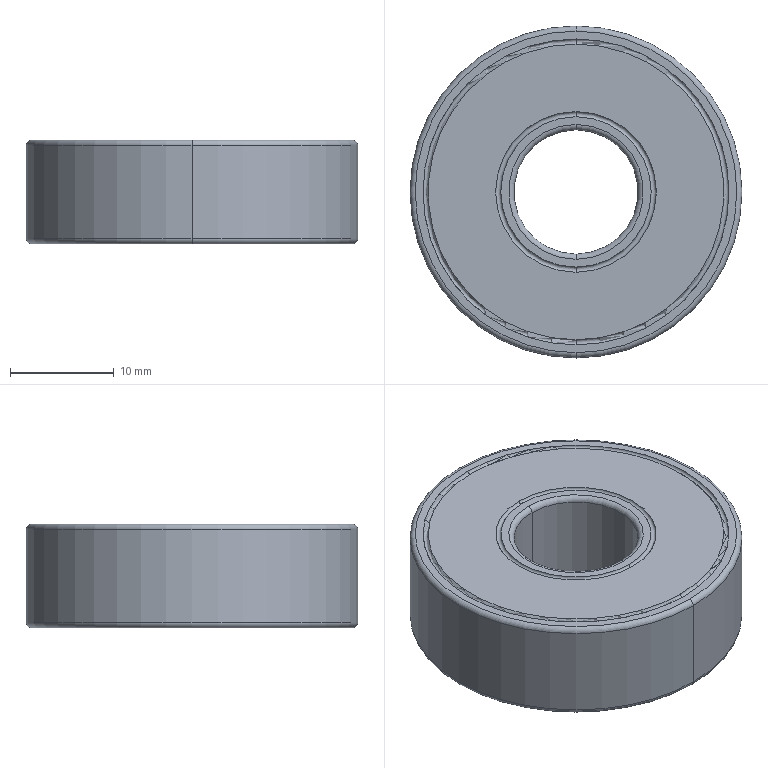Component | SolidWorks | --MA18S200416201Bearing-2 | 1 solid | 26 faces | box 32 x 32 x 10 mm | volume 6870 mm3 | torus 16 | plane 6 | cylinder 4 | commonest cylinder face diameters 12 x2 32 x2
build123d program:
from build123d import *

# Parameters (mm, degrees)
FILLET1_R = 0.5


with BuildPart() as part:
    # Sketch2 → Revolve1 (revolve)
    with BuildSketch(Plane.XY, mode=Mode.PRIVATE) as revolve1_sk:
        with BuildLine():
            Line((7.25, 10), (6, 10))
            Line((6, 10), (6, 0))
            Line((6, 0), (7.25, 0))
            ThreePointArc((7.25, 0), (7.5, 0.25), (7.75, 0))
            Line((7.75, 0), (14.25, 0))
            ThreePointArc((14.25, 0), (14.5, 0.25), (14.75, 0))
            Line((14.75, 0), (16, 0))
            Line((16, 0), (16, 10))
            Line((16, 10), (14.75, 10))
            ThreePointArc((14.75, 10), (14.5, 9.75), (14.25, 10))
            Line((14.25, 10), (7.75, 10))
            ThreePointArc((7.75, 10), (7.5, 9.75), (7.25, 10))
        make_face()
    revolve(revolve1_sk.sketch.rotate(Axis((0, 0, 0), (0, 1, 0)), 90), axis=Axis((0, 0, 0), (0, 1, 0)))

    # Fillet1
    fillet1_edges = [part.edges().sort_by_distance(p)[0] for p in [
        (0, 0, 6),
        (0, 10, 6),
        (0, 10, 16),
        (0, 0, 16),
    ]]
    fillet(fillet1_edges, radius=FILLET1_R)


solid = part.part

# Placed as in the assembly
solid = solid.moved(Location((72.885, -33.301, 50.5), (90, 0, 0)))
STEP:
#1=COLOUR_RGB('',0.7922,0.8196,0.9333);
#2=FILL_AREA_STYLE_COLOUR('',#1);
#3=FILL_AREA_STYLE('',(#2));
#4=SURFACE_STYLE_FILL_AREA(#3);
#5=SURFACE_SIDE_STYLE('',(#4));
#6=SURFACE_STYLE_USAGE(.BOTH.,#5);
#7=PRESENTATION_STYLE_ASSIGNMENT((#6));
#8=CARTESIAN_POINT('',(2.869,-1.941,2.008));
#9=VERTEX_POINT('',#8);
#10=CARTESIAN_POINT('',(2.869,-0.6811,2.008));
#11=VERTEX_POINT('',#10);
#12=CARTESIAN_POINT('',(2.869,-1.311,2.008));
#13=DIRECTION('',(0.,0.,1.));
#14=DIRECTION('',(0.,1.,0.));
#15=AXIS2_PLACEMENT_3D('',#12,#13,#14);
#16=CIRCLE('',#15,0.6299);
#17=EDGE_CURVE('',#9,#11,#16,.T.);
#18=ORIENTED_EDGE('',*,*,#17,.F.);
#19=CARTESIAN_POINT('',(2.869,-1.921,1.988));
#20=VERTEX_POINT('',#19);
#21=CARTESIAN_POINT('',(2.869,-1.921,2.008));
#22=DIRECTION('',(1.,0.,0.));
#23=DIRECTION('',(0.,1.,0.));
#24=AXIS2_PLACEMENT_3D('',#21,#22,#23);
#25=CIRCLE('',#24,0.01969);
#26=EDGE_CURVE('',#9,#20,#25,.T.);
#27=ORIENTED_EDGE('',*,*,#26,.T.);
#28=CARTESIAN_POINT('',(2.869,-0.7008,1.988));
#29=VERTEX_POINT('',#28);
#30=CARTESIAN_POINT('',(2.869,-1.311,1.988));
#31=DIRECTION('',(0.,0.,-1.));
#32=DIRECTION('',(0.,1.,0.));
#33=AXIS2_PLACEMENT_3D('',#30,#31,#32);
#34=CIRCLE('',#33,0.6102);
#35=EDGE_CURVE('',#29,#20,#34,.T.);
#36=ORIENTED_EDGE('',*,*,#35,.F.);
#37=CARTESIAN_POINT('',(2.869,-0.7008,2.008));
#38=DIRECTION('',(-1.,0.,0.));
#39=DIRECTION('',(0.,0.,1.));
#40=AXIS2_PLACEMENT_3D('',#37,#38,#39);
#41=CIRCLE('',#40,0.01969);
#42=EDGE_CURVE('',#11,#29,#41,.T.);
#43=ORIENTED_EDGE('',*,*,#42,.F.);
#44=EDGE_LOOP('',(#18,#27,#36,#43));
#45=FACE_OUTER_BOUND('',#44,.T.);
#46=CARTESIAN_POINT('',(2.869,-1.311,2.008));
#47=DIRECTION('',(0.,0.,-1.));
#48=DIRECTION('',(0.,1.,0.));
#49=AXIS2_PLACEMENT_3D('',#46,#47,#48);
#50=TOROIDAL_SURFACE('',#49,0.6102,0.01969);
#51=ADVANCED_FACE('',(#45),#50,.T.);
#52=CARTESIAN_POINT('',(2.869,-0.6811,2.362));
#53=VERTEX_POINT('',#52);
#54=CARTESIAN_POINT('',(2.869,-1.941,2.362));
#55=VERTEX_POINT('',#54);
#56=CARTESIAN_POINT('',(2.869,-1.311,2.362));
#57=DIRECTION('',(0.,0.,-1.));
#58=DIRECTION('',(0.,-1.,0.));
#59=AXIS2_PLACEMENT_3D('',#56,#57,#58);
#60=CIRCLE('',#59,0.6299);
#61=EDGE_CURVE('',#53,#55,#60,.T.);
#62=ORIENTED_EDGE('',*,*,#61,.F.);
#63=CARTESIAN_POINT('',(2.869,-0.7008,2.382));
#64=VERTEX_POINT('',#63);
#65=CARTESIAN_POINT('',(2.869,-0.7008,2.362));
#66=DIRECTION('',(1.,-0.,0.));
#67=DIRECTION('',(0.,1.,0.));
#68=AXIS2_PLACEMENT_3D('',#65,#66,#67);
#69=CIRCLE('',#68,0.01969);
#70=EDGE_CURVE('',#53,#64,#69,.T.);
#71=ORIENTED_EDGE('',*,*,#70,.T.);
#72=CARTESIAN_POINT('',(2.869,-1.921,2.382));
#73=VERTEX_POINT('',#72);
#74=CARTESIAN_POINT('',(2.869,-1.311,2.382));
#75=DIRECTION('',(0.,0.,1.));
#76=DIRECTION('',(0.,-1.,0.));
#77=AXIS2_PLACEMENT_3D('',#74,#75,#76);
#78=CIRCLE('',#77,0.6102);
#79=EDGE_CURVE('',#73,#64,#78,.T.);
#80=ORIENTED_EDGE('',*,*,#79,.F.);
#81=CARTESIAN_POINT('',(2.869,-1.921,2.362));
#82=DIRECTION('',(-1.,0.,0.));
#83=DIRECTION('',(0.,0.,1.));
#84=AXIS2_PLACEMENT_3D('',#81,#82,#83);
#85=CIRCLE('',#84,0.01969);
#86=EDGE_CURVE('',#55,#73,#85,.T.);
#87=ORIENTED_EDGE('',*,*,#86,.F.);
#88=EDGE_LOOP('',(#62,#71,#80,#87));
#89=FACE_OUTER_BOUND('',#88,.T.);
#90=CARTESIAN_POINT('',(2.869,-1.311,2.362));
#91=DIRECTION('',(0.,0.,1.));
#92=DIRECTION('',(0.,-1.,0.));
#93=AXIS2_PLACEMENT_3D('',#90,#91,#92);
#94=TOROIDAL_SURFACE('',#93,0.6102,0.01969);
#95=ADVANCED_FACE('',(#89),#94,.T.);
#96=CARTESIAN_POINT('',(2.869,-1.567,1.988));
#97=VERTEX_POINT('',#96);
#98=CARTESIAN_POINT('',(2.869,-1.055,1.988));
#99=VERTEX_POINT('',#98);
#100=CARTESIAN_POINT('',(2.869,-1.311,1.988));
#101=DIRECTION('',(0.,0.,1.));
#102=DIRECTION('',(0.,1.,0.));
#103=AXIS2_PLACEMENT_3D('',#100,#101,#102);
#104=CIRCLE('',#103,0.2559);
#105=EDGE_CURVE('',#97,#99,#104,.T.);
#106=ORIENTED_EDGE('',*,*,#105,.F.);
#107=CARTESIAN_POINT('',(2.869,-1.547,2.008));
#108=VERTEX_POINT('',#107);
#109=CARTESIAN_POINT('',(2.869,-1.567,2.008));
#110=DIRECTION('',(1.,0.,0.));
#111=DIRECTION('',(0.,1.,0.));
#112=AXIS2_PLACEMENT_3D('',#109,#110,#111);
#113=CIRCLE('',#112,0.01969);
#114=EDGE_CURVE('',#97,#108,#113,.T.);
#115=ORIENTED_EDGE('',*,*,#114,.T.);
#116=CARTESIAN_POINT('',(2.869,-1.075,2.008));
#117=VERTEX_POINT('',#116);
#118=CARTESIAN_POINT('',(2.869,-1.311,2.008));
#119=DIRECTION('',(0.,0.,-1.));
#120=DIRECTION('',(0.,1.,0.));
#121=AXIS2_PLACEMENT_3D('',#118,#119,#120);
#122=CIRCLE('',#121,0.2362);
#123=EDGE_CURVE('',#117,#108,#122,.T.);
#124=ORIENTED_EDGE('',*,*,#123,.F.);
#125=CARTESIAN_POINT('',(2.869,-1.055,2.008));
#126=DIRECTION('',(-1.,0.,0.));
#127=DIRECTION('',(0.,0.,1.));
#128=AXIS2_PLACEMENT_3D('',#125,#126,#127);
#129=CIRCLE('',#128,0.01969);
#130=EDGE_CURVE('',#99,#117,#129,.T.);
#131=ORIENTED_EDGE('',*,*,#130,.F.);
#132=EDGE_LOOP('',(#106,#115,#124,#131));
#133=FACE_OUTER_BOUND('',#132,.T.);
#134=CARTESIAN_POINT('',(2.869,-1.311,2.008));
#135=DIRECTION('',(0.,0.,-1.));
#136=DIRECTION('',(0.,1.,0.));
#137=AXIS2_PLACEMENT_3D('',#134,#135,#136);
#138=TOROIDAL_SURFACE('',#137,0.2559,0.01969);
#139=ADVANCED_FACE('',(#133),#138,.T.);
#140=CARTESIAN_POINT('',(2.869,-1.055,2.382));
#141=VERTEX_POINT('',#140);
#142=CARTESIAN_POINT('',(2.869,-1.567,2.382));
#143=VERTEX_POINT('',#142);
#144=CARTESIAN_POINT('',(2.869,-1.311,2.382));
#145=DIRECTION('',(0.,0.,-1.));
#146=DIRECTION('',(0.,-1.,0.));
#147=AXIS2_PLACEMENT_3D('',#144,#145,#146);
#148=CIRCLE('',#147,0.2559);
#149=EDGE_CURVE('',#141,#143,#148,.T.);
#150=ORIENTED_EDGE('',*,*,#149,.F.);
#151=CARTESIAN_POINT('',(2.869,-1.075,2.362));
#152=VERTEX_POINT('',#151);
#153=CARTESIAN_POINT('',(2.869,-1.055,2.362));
#154=DIRECTION('',(1.,-0.,0.));
#155=DIRECTION('',(0.,1.,0.));
#156=AXIS2_PLACEMENT_3D('',#153,#154,#155);
#157=CIRCLE('',#156,0.01969);
#158=EDGE_CURVE('',#141,#152,#157,.T.);
#159=ORIENTED_EDGE('',*,*,#158,.T.);
#160=CARTESIAN_POINT('',(2.869,-1.547,2.362));
#161=VERTEX_POINT('',#160);
#162=CARTESIAN_POINT('',(2.869,-1.311,2.362));
#163=DIRECTION('',(0.,0.,1.));
#164=DIRECTION('',(0.,-1.,0.));
#165=AXIS2_PLACEMENT_3D('',#162,#163,#164);
#166=CIRCLE('',#165,0.2362);
#167=EDGE_CURVE('',#161,#152,#166,.T.);
#168=ORIENTED_EDGE('',*,*,#167,.F.);
#169=CARTESIAN_POINT('',(2.869,-1.567,2.362));
#170=DIRECTION('',(-1.,0.,0.));
#171=DIRECTION('',(0.,0.,1.));
#172=AXIS2_PLACEMENT_3D('',#169,#170,#171);
#173=CIRCLE('',#172,0.01969);
#174=EDGE_CURVE('',#143,#161,#173,.T.);
#175=ORIENTED_EDGE('',*,*,#174,.F.);
#176=EDGE_LOOP('',(#150,#159,#168,#175));
#177=FACE_OUTER_BOUND('',#176,.T.);
#178=CARTESIAN_POINT('',(2.869,-1.311,2.362));
#179=DIRECTION('',(0.,0.,1.));
#180=DIRECTION('',(0.,-1.,0.));
#181=AXIS2_PLACEMENT_3D('',#178,#179,#180);
#182=TOROIDAL_SURFACE('',#181,0.2559,0.01969);
#183=ADVANCED_FACE('',(#177),#182,.T.);
#184=CARTESIAN_POINT('',(2.869,-0.75,2.382));
#185=VERTEX_POINT('',#184);
#186=CARTESIAN_POINT('',(2.869,-1.872,2.382));
#187=VERTEX_POINT('',#186);
#188=CARTESIAN_POINT('',(2.869,-1.311,2.382));
#189=DIRECTION('',(0.,0.,1.));
#190=DIRECTION('',(0.,-1.,0.));
#191=AXIS2_PLACEMENT_3D('',#188,#189,#190);
#192=CIRCLE('',#191,0.561);
#193=EDGE_CURVE('',#185,#187,#192,.T.);
#194=ORIENTED_EDGE('',*,*,#193,.F.);
#195=CARTESIAN_POINT('',(2.869,-0.7304,2.382));
#196=VERTEX_POINT('',#195);
#197=CARTESIAN_POINT('',(2.869,-0.7402,2.382));
#198=DIRECTION('',(1.,-0.,0.));
#199=DIRECTION('',(0.,1.,0.));
#200=AXIS2_PLACEMENT_3D('',#197,#198,#199);
#201=CIRCLE('',#200,0.009843);
#202=EDGE_CURVE('',#185,#196,#201,.T.);
#203=ORIENTED_EDGE('',*,*,#202,.T.);
#204=CARTESIAN_POINT('',(2.869,-1.892,2.382));
#205=VERTEX_POINT('',#204);
#206=CARTESIAN_POINT('',(2.869,-1.311,2.382));
#207=DIRECTION('',(0.,0.,1.));
#208=DIRECTION('',(0.,-1.,0.));
#209=AXIS2_PLACEMENT_3D('',#206,#207,#208);
#210=CIRCLE('',#209,0.5807);
#211=EDGE_CURVE('',#196,#205,#210,.T.);
#212=ORIENTED_EDGE('',*,*,#211,.T.);
#213=CARTESIAN_POINT('',(2.869,-1.882,2.382));
#214=DIRECTION('',(-1.,0.,0.));
#215=DIRECTION('',(0.,0.,1.));
#216=AXIS2_PLACEMENT_3D('',#213,#214,#215);
#217=CIRCLE('',#216,0.009843);
#218=EDGE_CURVE('',#187,#205,#217,.T.);
#219=ORIENTED_EDGE('',*,*,#218,.F.);
#220=EDGE_LOOP('',(#194,#203,#212,#219));
#221=FACE_OUTER_BOUND('',#220,.T.);
#222=CARTESIAN_POINT('',(2.869,-1.311,2.382));
#223=DIRECTION('',(0.,0.,1.));
#224=DIRECTION('',(0.,-1.,0.));
#225=AXIS2_PLACEMENT_3D('',#222,#223,#224);
#226=TOROIDAL_SURFACE('',#225,0.5709,0.009843);
#227=ADVANCED_FACE('',(#221),#226,.F.);
#228=CARTESIAN_POINT('',(2.869,-1.026,2.382));
#229=VERTEX_POINT('',#228);
#230=CARTESIAN_POINT('',(2.869,-1.597,2.382));
#231=VERTEX_POINT('',#230);
#232=CARTESIAN_POINT('',(2.869,-1.311,2.382));
#233=DIRECTION('',(0.,0.,1.));
#234=DIRECTION('',(0.,-1.,0.));
#235=AXIS2_PLACEMENT_3D('',#232,#233,#234);
#236=CIRCLE('',#235,0.2854);
#237=EDGE_CURVE('',#229,#231,#236,.T.);
#238=ORIENTED_EDGE('',*,*,#237,.F.);
#239=CARTESIAN_POINT('',(2.869,-1.006,2.382));
#240=VERTEX_POINT('',#239);
#241=CARTESIAN_POINT('',(2.869,-1.016,2.382));
#242=DIRECTION('',(1.,-0.,0.));
#243=DIRECTION('',(0.,1.,0.));
#244=AXIS2_PLACEMENT_3D('',#241,#242,#243);
#245=CIRCLE('',#244,0.009843);
#246=EDGE_CURVE('',#229,#240,#245,.T.);
#247=ORIENTED_EDGE('',*,*,#246,.T.);
#248=CARTESIAN_POINT('',(2.869,-1.616,2.382));
#249=VERTEX_POINT('',#248);
#250=CARTESIAN_POINT('',(2.869,-1.311,2.382));
#251=DIRECTION('',(0.,0.,1.));
#252=DIRECTION('',(0.,-1.,0.));
#253=AXIS2_PLACEMENT_3D('',#250,#251,#252);
#254=CIRCLE('',#253,0.3051);
#255=EDGE_CURVE('',#240,#249,#254,.T.);
#256=ORIENTED_EDGE('',*,*,#255,.T.);
#257=CARTESIAN_POINT('',(2.869,-1.606,2.382));
#258=DIRECTION('',(-1.,0.,0.));
#259=DIRECTION('',(0.,0.,1.));
#260=AXIS2_PLACEMENT_3D('',#257,#258,#259);
#261=CIRCLE('',#260,0.009843);
#262=EDGE_CURVE('',#231,#249,#261,.T.);
#263=ORIENTED_EDGE('',*,*,#262,.F.);
#264=EDGE_LOOP('',(#238,#247,#256,#263));
#265=FACE_OUTER_BOUND('',#264,.T.);
#266=CARTESIAN_POINT('',(2.869,-1.311,2.382));
#267=DIRECTION('',(0.,0.,1.));
#268=DIRECTION('',(0.,-1.,0.));
#269=AXIS2_PLACEMENT_3D('',#266,#267,#268);
#270=TOROIDAL_SURFACE('',#269,0.2953,0.009843);
#271=ADVANCED_FACE('',(#265),#270,.F.);
#272=CARTESIAN_POINT('',(2.869,-1.311,2.008));
#273=DIRECTION('',(0.,0.,-1.));
#274=DIRECTION('',(0.,1.,0.));
#275=AXIS2_PLACEMENT_3D('',#272,#273,#274);
#276=CIRCLE('',#275,0.2362);
#277=EDGE_CURVE('',#108,#117,#276,.T.);
#278=ORIENTED_EDGE('',*,*,#277,.T.);
#279=CARTESIAN_POINT('',(2.869,-1.075,2.382));
#280=DIRECTION('',(0.,0.,1.));
#281=VECTOR('',#280,39.37);
#282=LINE('',#279,#281);
#283=EDGE_CURVE('',#117,#152,#282,.T.);
#284=ORIENTED_EDGE('',*,*,#283,.T.);
#285=CARTESIAN_POINT('',(2.869,-1.311,2.362));
#286=DIRECTION('',(0.,0.,1.));
#287=DIRECTION('',(0.,-1.,0.));
#288=AXIS2_PLACEMENT_3D('',#285,#286,#287);
#289=CIRCLE('',#288,0.2362);
#290=EDGE_CURVE('',#152,#161,#289,.T.);
#291=ORIENTED_EDGE('',*,*,#290,.T.);
#292=CARTESIAN_POINT('',(2.869,-1.547,2.382));
#293=DIRECTION('',(0.,0.,1.));
#294=VECTOR('',#293,39.37);
#295=LINE('',#292,#294);
#296=EDGE_CURVE('',#108,#161,#295,.T.);
#297=ORIENTED_EDGE('',*,*,#296,.F.);
#298=EDGE_LOOP('',(#278,#284,#291,#297));
#299=FACE_OUTER_BOUND('',#298,.T.);
#300=CARTESIAN_POINT('',(2.869,-1.311,2.382));
#301=DIRECTION('',(0.,0.,1.));
#302=DIRECTION('',(0.,-1.,0.));
#303=AXIS2_PLACEMENT_3D('',#300,#301,#302);
#304=CYLINDRICAL_SURFACE('',#303,0.2362);
#305=ADVANCED_FACE('',(#299),#304,.F.);
#306=CARTESIAN_POINT('',(2.869,-1.006,1.988));
#307=VERTEX_POINT('',#306);
#308=CARTESIAN_POINT('',(2.869,-1.616,1.988));
#309=VERTEX_POINT('',#308);
#310=CARTESIAN_POINT('',(2.869,-1.311,1.988));
#311=DIRECTION('',(0.,0.,1.));
#312=DIRECTION('',(0.,-1.,0.));
#313=AXIS2_PLACEMENT_3D('',#310,#311,#312);
#314=CIRCLE('',#313,0.3051);
#315=EDGE_CURVE('',#307,#309,#314,.T.);
#316=ORIENTED_EDGE('',*,*,#315,.F.);
#317=CARTESIAN_POINT('',(2.869,-1.026,1.988));
#318=VERTEX_POINT('',#317);
#319=CARTESIAN_POINT('',(2.869,-1.016,1.988));
#320=DIRECTION('',(1.,-0.,0.));
#321=DIRECTION('',(0.,1.,0.));
#322=AXIS2_PLACEMENT_3D('',#319,#320,#321);
#323=CIRCLE('',#322,0.009843);
#324=EDGE_CURVE('',#307,#318,#323,.T.);
#325=ORIENTED_EDGE('',*,*,#324,.T.);
#326=CARTESIAN_POINT('',(2.869,-1.597,1.988));
#327=VERTEX_POINT('',#326);
#328=CARTESIAN_POINT('',(2.869,-1.311,1.988));
#329=DIRECTION('',(0.,0.,1.));
#330=DIRECTION('',(0.,-1.,0.));
#331=AXIS2_PLACEMENT_3D('',#328,#329,#330);
#332=CIRCLE('',#331,0.2854);
#333=EDGE_CURVE('',#318,#327,#332,.T.);
#334=ORIENTED_EDGE('',*,*,#333,.T.);
#335=CARTESIAN_POINT('',(2.869,-1.606,1.988));
#336=DIRECTION('',(-1.,0.,0.));
#337=DIRECTION('',(0.,0.,1.));
#338=AXIS2_PLACEMENT_3D('',#335,#336,#337);
#339=CIRCLE('',#338,0.009843);
#340=EDGE_CURVE('',#309,#327,#339,.T.);
#341=ORIENTED_EDGE('',*,*,#340,.F.);
#342=EDGE_LOOP('',(#316,#325,#334,#341));
#343=FACE_OUTER_BOUND('',#342,.T.);
#344=CARTESIAN_POINT('',(2.869,-1.311,1.988));
#345=DIRECTION('',(0.,0.,1.));
#346=DIRECTION('',(0.,-1.,0.));
#347=AXIS2_PLACEMENT_3D('',#344,#345,#346);
#348=TOROIDAL_SURFACE('',#347,0.2953,0.009843);
#349=ADVANCED_FACE('',(#343),#348,.F.);
#350=CARTESIAN_POINT('',(2.869,-0.7304,1.988));
#351=VERTEX_POINT('',#350);
#352=CARTESIAN_POINT('',(2.869,-1.892,1.988));
#353=VERTEX_POINT('',#352);
#354=CARTESIAN_POINT('',(2.869,-1.311,1.988));
#355=DIRECTION('',(0.,0.,1.));
#356=DIRECTION('',(0.,-1.,0.));
#357=AXIS2_PLACEMENT_3D('',#354,#355,#356);
#358=CIRCLE('',#357,0.5807);
#359=EDGE_CURVE('',#351,#353,#358,.T.);
#360=ORIENTED_EDGE('',*,*,#359,.F.);
#361=CARTESIAN_POINT('',(2.869,-0.75,1.988));
#362=VERTEX_POINT('',#361);
#363=CARTESIAN_POINT('',(2.869,-0.7402,1.988));
#364=DIRECTION('',(1.,-0.,0.));
#365=DIRECTION('',(0.,1.,0.));
#366=AXIS2_PLACEMENT_3D('',#363,#364,#365);
#367=CIRCLE('',#366,0.009843);
#368=EDGE_CURVE('',#351,#362,#367,.T.);
#369=ORIENTED_EDGE('',*,*,#368,.T.);
#370=CARTESIAN_POINT('',(2.869,-1.872,1.988));
#371=VERTEX_POINT('',#370);
#372=CARTESIAN_POINT('',(2.869,-1.311,1.988));
#373=DIRECTION('',(0.,0.,1.));
#374=DIRECTION('',(0.,-1.,0.));
#375=AXIS2_PLACEMENT_3D('',#372,#373,#374);
#376=CIRCLE('',#375,0.561);
#377=EDGE_CURVE('',#362,#371,#376,.T.);
#378=ORIENTED_EDGE('',*,*,#377,.T.);
#379=CARTESIAN_POINT('',(2.869,-1.882,1.988));
#380=DIRECTION('',(-1.,0.,0.));
#381=DIRECTION('',(0.,0.,1.));
#382=AXIS2_PLACEMENT_3D('',#379,#380,#381);
#383=CIRCLE('',#382,0.009843);
#384=EDGE_CURVE('',#353,#371,#383,.T.);
#385=ORIENTED_EDGE('',*,*,#384,.F.);
#386=EDGE_LOOP('',(#360,#369,#378,#385));
#387=FACE_OUTER_BOUND('',#386,.T.);
#388=CARTESIAN_POINT('',(2.869,-1.311,1.988));
#389=DIRECTION('',(0.,0.,1.));
#390=DIRECTION('',(0.,-1.,0.));
#391=AXIS2_PLACEMENT_3D('',#388,#389,#390);
#392=TOROIDAL_SURFACE('',#391,0.5709,0.009843);
#393=ADVANCED_FACE('',(#387),#392,.F.);
#394=ORIENTED_EDGE('',*,*,#17,.T.);
#395=CARTESIAN_POINT('',(2.869,-0.6811,2.382));
#396=DIRECTION('',(0.,0.,1.));
#397=VECTOR('',#396,39.37);
#398=LINE('',#395,#397);
#399=EDGE_CURVE('',#11,#53,#398,.T.);
#400=ORIENTED_EDGE('',*,*,#399,.T.);
#401=ORIENTED_EDGE('',*,*,#61,.T.);
#402=CARTESIAN_POINT('',(2.869,-1.941,2.382));
#403=DIRECTION('',(0.,0.,1.));
#404=VECTOR('',#403,39.37);
#405=LINE('',#402,#404);
#406=EDGE_CURVE('',#9,#55,#405,.T.);
#407=ORIENTED_EDGE('',*,*,#406,.F.);
#408=EDGE_LOOP('',(#394,#400,#401,#407));
#409=FACE_OUTER_BOUND('',#408,.T.);
#410=CARTESIAN_POINT('',(2.869,-1.311,2.382));
#411=DIRECTION('',(0.,0.,1.));
#412=DIRECTION('',(0.,-1.,0.));
#413=AXIS2_PLACEMENT_3D('',#410,#411,#412);
#414=CYLINDRICAL_SURFACE('',#413,0.6299);
#415=ADVANCED_FACE('',(#409),#414,.T.);
#416=ORIENTED_EDGE('',*,*,#399,.F.);
#417=CARTESIAN_POINT('',(2.869,-1.311,2.008));
#418=DIRECTION('',(0.,0.,1.));
#419=DIRECTION('',(0.,1.,0.));
#420=AXIS2_PLACEMENT_3D('',#417,#418,#419);
#421=CIRCLE('',#420,0.6299);
#422=EDGE_CURVE('',#11,#9,#421,.T.);
#423=ORIENTED_EDGE('',*,*,#422,.T.);
#424=ORIENTED_EDGE('',*,*,#406,.T.);
#425=CARTESIAN_POINT('',(2.869,-1.311,2.362));
#426=DIRECTION('',(0.,0.,-1.));
#427=DIRECTION('',(0.,-1.,0.));
#428=AXIS2_PLACEMENT_3D('',#425,#426,#427);
#429=CIRCLE('',#428,0.6299);
#430=EDGE_CURVE('',#55,#53,#429,.T.);
#431=ORIENTED_EDGE('',*,*,#430,.T.);
#432=EDGE_LOOP('',(#416,#423,#424,#431));
#433=FACE_OUTER_BOUND('',#432,.T.);
#434=CARTESIAN_POINT('',(2.869,-1.311,2.382));
#435=DIRECTION('',(0.,0.,1.));
#436=DIRECTION('',(0.,-1.,0.));
#437=AXIS2_PLACEMENT_3D('',#434,#435,#436);
#438=CYLINDRICAL_SURFACE('',#437,0.6299);
#439=ADVANCED_FACE('',(#433),#438,.T.);
#440=ORIENTED_EDGE('',*,*,#35,.T.);
#441=CARTESIAN_POINT('',(2.869,-1.311,1.988));
#442=DIRECTION('',(0.,0.,-1.));
#443=DIRECTION('',(0.,1.,0.));
#444=AXIS2_PLACEMENT_3D('',#441,#442,#443);
#445=CIRCLE('',#444,0.6102);
#446=EDGE_CURVE('',#20,#29,#445,.T.);
#447=ORIENTED_EDGE('',*,*,#446,.T.);
#448=EDGE_LOOP('',(#440,#447));
#449=FACE_OUTER_BOUND('',#448,.T.);
#450=CARTESIAN_POINT('',(2.869,-1.311,1.988));
#451=DIRECTION('',(0.,0.,1.));
#452=DIRECTION('',(0.,-1.,0.));
#453=AXIS2_PLACEMENT_3D('',#450,#451,#452);
#454=CIRCLE('',#453,0.5807);
#455=EDGE_CURVE('',#353,#351,#454,.T.);
#456=ORIENTED_EDGE('',*,*,#455,.T.);
#457=ORIENTED_EDGE('',*,*,#359,.T.);
#458=EDGE_LOOP('',(#456,#457));
#459=FACE_BOUND('',#458,.T.);
#460=CARTESIAN_POINT('',(3.499,-1.311,1.988));
#461=DIRECTION('',(0.,0.,-1.));
#462=DIRECTION('',(0.,1.,0.));
#463=AXIS2_PLACEMENT_3D('',#460,#461,#462);
#464=PLANE('',#463);
#465=ADVANCED_FACE('',(#449,#459),#464,.T.);
#466=ORIENTED_EDGE('',*,*,#368,.F.);
#467=ORIENTED_EDGE('',*,*,#455,.F.);
#468=ORIENTED_EDGE('',*,*,#384,.T.);
#469=CARTESIAN_POINT('',(2.869,-1.311,1.988));
#470=DIRECTION('',(0.,0.,1.));
#471=DIRECTION('',(0.,-1.,0.));
#472=AXIS2_PLACEMENT_3D('',#469,#470,#471);
#473=CIRCLE('',#472,0.561);
#474=EDGE_CURVE('',#371,#362,#473,.T.);
#475=ORIENTED_EDGE('',*,*,#474,.T.);
#476=EDGE_LOOP('',(#466,#467,#468,#475));
#477=FACE_OUTER_BOUND('',#476,.T.);
#478=CARTESIAN_POINT('',(2.869,-1.311,1.988));
#479=DIRECTION('',(0.,0.,1.));
#480=DIRECTION('',(0.,-1.,0.));
#481=AXIS2_PLACEMENT_3D('',#478,#479,#480);
#482=TOROIDAL_SURFACE('',#481,0.5709,0.009843);
#483=ADVANCED_FACE('',(#477),#482,.F.);
#484=CARTESIAN_POINT('',(2.869,-1.311,1.988));
#485=DIRECTION('',(0.,0.,1.));
#486=DIRECTION('',(0.,-1.,0.));
#487=AXIS2_PLACEMENT_3D('',#484,#485,#486);
#488=CIRCLE('',#487,0.3051);
#489=EDGE_CURVE('',#309,#307,#488,.T.);
#490=ORIENTED_EDGE('',*,*,#489,.T.);
#491=ORIENTED_EDGE('',*,*,#315,.T.);
#492=EDGE_LOOP('',(#490,#491));
#493=FACE_BOUND('',#492,.T.);
#494=ORIENTED_EDGE('',*,*,#474,.F.);
#495=ORIENTED_EDGE('',*,*,#377,.F.);
#496=EDGE_LOOP('',(#494,#495));
#497=FACE_OUTER_BOUND('',#496,.T.);
#498=CARTESIAN_POINT('',(3.431,-1.311,1.988));
#499=DIRECTION('',(0.,0.,-1.));
#500=DIRECTION('',(0.,1.,0.));
#501=AXIS2_PLACEMENT_3D('',#498,#499,#500);
#502=PLANE('',#501);
#503=ADVANCED_FACE('',(#493,#497),#502,.T.);
#504=ORIENTED_EDGE('',*,*,#324,.F.);
#505=ORIENTED_EDGE('',*,*,#489,.F.);
#506=ORIENTED_EDGE('',*,*,#340,.T.);
#507=CARTESIAN_POINT('',(2.869,-1.311,1.988));
#508=DIRECTION('',(0.,0.,1.));
#509=DIRECTION('',(0.,-1.,0.));
#510=AXIS2_PLACEMENT_3D('',#507,#508,#509);
#511=CIRCLE('',#510,0.2854);
#512=EDGE_CURVE('',#327,#318,#511,.T.);
#513=ORIENTED_EDGE('',*,*,#512,.T.);
#514=EDGE_LOOP('',(#504,#505,#506,#513));
#515=FACE_OUTER_BOUND('',#514,.T.);
#516=CARTESIAN_POINT('',(2.869,-1.311,1.988));
#517=DIRECTION('',(0.,0.,1.));
#518=DIRECTION('',(0.,-1.,0.));
#519=AXIS2_PLACEMENT_3D('',#516,#517,#518);
#520=TOROIDAL_SURFACE('',#519,0.2953,0.009843);
#521=ADVANCED_FACE('',(#515),#520,.F.);
#522=CARTESIAN_POINT('',(2.869,-1.311,1.988));
#523=DIRECTION('',(0.,0.,1.));
#524=DIRECTION('',(0.,1.,0.));
#525=AXIS2_PLACEMENT_3D('',#522,#523,#524);
#526=CIRCLE('',#525,0.2559);
#527=EDGE_CURVE('',#99,#97,#526,.T.);
#528=ORIENTED_EDGE('',*,*,#527,.T.);
#529=ORIENTED_EDGE('',*,*,#105,.T.);
#530=EDGE_LOOP('',(#528,#529));
#531=FACE_BOUND('',#530,.T.);
#532=ORIENTED_EDGE('',*,*,#512,.F.);
#533=ORIENTED_EDGE('',*,*,#333,.F.);
#534=EDGE_LOOP('',(#532,#533));
#535=FACE_OUTER_BOUND('',#534,.T.);
#536=CARTESIAN_POINT('',(3.155,-1.311,1.988));
#537=DIRECTION('',(0.,0.,-1.));
#538=DIRECTION('',(0.,1.,0.));
#539=AXIS2_PLACEMENT_3D('',#536,#537,#538);
#540=PLANE('',#539);
#541=ADVANCED_FACE('',(#531,#535),#540,.T.);
#542=ORIENTED_EDGE('',*,*,#283,.F.);
#543=ORIENTED_EDGE('',*,*,#123,.T.);
#544=ORIENTED_EDGE('',*,*,#296,.T.);
#545=ORIENTED_EDGE('',*,*,#167,.T.);
#546=EDGE_LOOP('',(#542,#543,#544,#545));
#547=FACE_OUTER_BOUND('',#546,.T.);
#548=CARTESIAN_POINT('',(2.869,-1.311,2.382));
#549=DIRECTION('',(0.,0.,1.));
#550=DIRECTION('',(0.,-1.,0.));
#551=AXIS2_PLACEMENT_3D('',#548,#549,#550);
#552=CYLINDRICAL_SURFACE('',#551,0.2362);
#553=ADVANCED_FACE('',(#547),#552,.F.);
#554=CARTESIAN_POINT('',(2.869,-1.311,2.382));
#555=DIRECTION('',(0.,0.,-1.));
#556=DIRECTION('',(0.,-1.,0.));
#557=AXIS2_PLACEMENT_3D('',#554,#555,#556);
#558=CIRCLE('',#557,0.2559);
#559=EDGE_CURVE('',#143,#141,#558,.T.);
#560=ORIENTED_EDGE('',*,*,#559,.T.);
#561=ORIENTED_EDGE('',*,*,#149,.T.);
#562=EDGE_LOOP('',(#560,#561));
#563=FACE_BOUND('',#562,.T.);
#564=CARTESIAN_POINT('',(2.869,-1.311,2.382));
#565=DIRECTION('',(0.,0.,1.));
#566=DIRECTION('',(0.,-1.,0.));
#567=AXIS2_PLACEMENT_3D('',#564,#565,#566);
#568=CIRCLE('',#567,0.2854);
#569=EDGE_CURVE('',#231,#229,#568,.T.);
#570=ORIENTED_EDGE('',*,*,#569,.T.);
#571=ORIENTED_EDGE('',*,*,#237,.T.);
#572=EDGE_LOOP('',(#570,#571));
#573=FACE_OUTER_BOUND('',#572,.T.);
#574=CARTESIAN_POINT('',(3.155,-1.311,2.382));
#575=DIRECTION('',(0.,0.,1.));
#576=DIRECTION('',(0.,-1.,0.));
#577=AXIS2_PLACEMENT_3D('',#574,#575,#576);
#578=PLANE('',#577);
#579=ADVANCED_FACE('',(#563,#573),#578,.T.);
#580=ORIENTED_EDGE('',*,*,#246,.F.);
#581=ORIENTED_EDGE('',*,*,#569,.F.);
#582=ORIENTED_EDGE('',*,*,#262,.T.);
#583=CARTESIAN_POINT('',(2.869,-1.311,2.382));
#584=DIRECTION('',(0.,0.,1.));
#585=DIRECTION('',(0.,-1.,0.));
#586=AXIS2_PLACEMENT_3D('',#583,#584,#585);
#587=CIRCLE('',#586,0.3051);
#588=EDGE_CURVE('',#249,#240,#587,.T.);
#589=ORIENTED_EDGE('',*,*,#588,.T.);
#590=EDGE_LOOP('',(#580,#581,#582,#589));
#591=FACE_OUTER_BOUND('',#590,.T.);
#592=CARTESIAN_POINT('',(2.869,-1.311,2.382));
#593=DIRECTION('',(0.,0.,1.));
#594=DIRECTION('',(0.,-1.,0.));
#595=AXIS2_PLACEMENT_3D('',#592,#593,#594);
#596=TOROIDAL_SURFACE('',#595,0.2953,0.009843);
#597=ADVANCED_FACE('',(#591),#596,.F.);
#598=CARTESIAN_POINT('',(2.869,-1.311,2.382));
#599=DIRECTION('',(0.,0.,1.));
#600=DIRECTION('',(0.,-1.,0.));
#601=AXIS2_PLACEMENT_3D('',#598,#599,#600);
#602=CIRCLE('',#601,0.561);
#603=EDGE_CURVE('',#187,#185,#602,.T.);
#604=ORIENTED_EDGE('',*,*,#603,.T.);
#605=ORIENTED_EDGE('',*,*,#193,.T.);
#606=EDGE_LOOP('',(#604,#605));
#607=FACE_OUTER_BOUND('',#606,.T.);
#608=ORIENTED_EDGE('',*,*,#588,.F.);
#609=ORIENTED_EDGE('',*,*,#255,.F.);
#610=EDGE_LOOP('',(#608,#609));
#611=FACE_BOUND('',#610,.T.);
#612=CARTESIAN_POINT('',(3.431,-1.311,2.382));
#613=DIRECTION('',(0.,0.,1.));
#614=DIRECTION('',(0.,-1.,0.));
#615=AXIS2_PLACEMENT_3D('',#612,#613,#614);
#616=PLANE('',#615);
#617=ADVANCED_FACE('',(#607,#611),#616,.T.);
#618=ORIENTED_EDGE('',*,*,#202,.F.);
#619=ORIENTED_EDGE('',*,*,#603,.F.);
#620=ORIENTED_EDGE('',*,*,#218,.T.);
#621=CARTESIAN_POINT('',(2.869,-1.311,2.382));
#622=DIRECTION('',(0.,0.,1.));
#623=DIRECTION('',(0.,-1.,0.));
#624=AXIS2_PLACEMENT_3D('',#621,#622,#623);
#625=CIRCLE('',#624,0.5807);
#626=EDGE_CURVE('',#205,#196,#625,.T.);
#627=ORIENTED_EDGE('',*,*,#626,.T.);
#628=EDGE_LOOP('',(#618,#619,#620,#627));
#629=FACE_OUTER_BOUND('',#628,.T.);
#630=CARTESIAN_POINT('',(2.869,-1.311,2.382));
#631=DIRECTION('',(0.,0.,1.));
#632=DIRECTION('',(0.,-1.,0.));
#633=AXIS2_PLACEMENT_3D('',#630,#631,#632);
#634=TOROIDAL_SURFACE('',#633,0.5709,0.009843);
#635=ADVANCED_FACE('',(#629),#634,.F.);
#636=ORIENTED_EDGE('',*,*,#79,.T.);
#637=CARTESIAN_POINT('',(2.869,-1.311,2.382));
#638=DIRECTION('',(0.,0.,1.));
#639=DIRECTION('',(0.,-1.,0.));
#640=AXIS2_PLACEMENT_3D('',#637,#638,#639);
#641=CIRCLE('',#640,0.6102);
#642=EDGE_CURVE('',#64,#73,#641,.T.);
#643=ORIENTED_EDGE('',*,*,#642,.T.);
#644=EDGE_LOOP('',(#636,#643));
#645=FACE_OUTER_BOUND('',#644,.T.);
#646=ORIENTED_EDGE('',*,*,#626,.F.);
#647=ORIENTED_EDGE('',*,*,#211,.F.);
#648=EDGE_LOOP('',(#646,#647));
#649=FACE_BOUND('',#648,.T.);
#650=CARTESIAN_POINT('',(3.499,-1.311,2.382));
#651=DIRECTION('',(0.,0.,1.));
#652=DIRECTION('',(0.,-1.,0.));
#653=AXIS2_PLACEMENT_3D('',#650,#651,#652);
#654=PLANE('',#653);
#655=ADVANCED_FACE('',(#645,#649),#654,.T.);
#656=ORIENTED_EDGE('',*,*,#158,.F.);
#657=ORIENTED_EDGE('',*,*,#559,.F.);
#658=ORIENTED_EDGE('',*,*,#174,.T.);
#659=ORIENTED_EDGE('',*,*,#290,.F.);
#660=EDGE_LOOP('',(#656,#657,#658,#659));
#661=FACE_OUTER_BOUND('',#660,.T.);
#662=CARTESIAN_POINT('',(2.869,-1.311,2.362));
#663=DIRECTION('',(0.,0.,1.));
#664=DIRECTION('',(0.,-1.,0.));
#665=AXIS2_PLACEMENT_3D('',#662,#663,#664);
#666=TOROIDAL_SURFACE('',#665,0.2559,0.01969);
#667=ADVANCED_FACE('',(#661),#666,.T.);
#668=ORIENTED_EDGE('',*,*,#114,.F.);
#669=ORIENTED_EDGE('',*,*,#527,.F.);
#670=ORIENTED_EDGE('',*,*,#130,.T.);
#671=ORIENTED_EDGE('',*,*,#277,.F.);
#672=EDGE_LOOP('',(#668,#669,#670,#671));
#673=FACE_OUTER_BOUND('',#672,.T.);
#674=CARTESIAN_POINT('',(2.869,-1.311,2.008));
#675=DIRECTION('',(0.,0.,-1.));
#676=DIRECTION('',(0.,1.,0.));
#677=AXIS2_PLACEMENT_3D('',#674,#675,#676);
#678=TOROIDAL_SURFACE('',#677,0.2559,0.01969);
#679=ADVANCED_FACE('',(#673),#678,.T.);
#680=ORIENTED_EDGE('',*,*,#70,.F.);
#681=ORIENTED_EDGE('',*,*,#430,.F.);
#682=ORIENTED_EDGE('',*,*,#86,.T.);
#683=ORIENTED_EDGE('',*,*,#642,.F.);
#684=EDGE_LOOP('',(#680,#681,#682,#683));
#685=FACE_OUTER_BOUND('',#684,.T.);
#686=CARTESIAN_POINT('',(2.869,-1.311,2.362));
#687=DIRECTION('',(0.,0.,1.));
#688=DIRECTION('',(0.,-1.,0.));
#689=AXIS2_PLACEMENT_3D('',#686,#687,#688);
#690=TOROIDAL_SURFACE('',#689,0.6102,0.01969);
#691=ADVANCED_FACE('',(#685),#690,.T.);
#692=ORIENTED_EDGE('',*,*,#26,.F.);
#693=ORIENTED_EDGE('',*,*,#422,.F.);
#694=ORIENTED_EDGE('',*,*,#42,.T.);
#695=ORIENTED_EDGE('',*,*,#446,.F.);
#696=EDGE_LOOP('',(#692,#693,#694,#695));
#697=FACE_OUTER_BOUND('',#696,.T.);
#698=CARTESIAN_POINT('',(2.869,-1.311,2.008));
#699=DIRECTION('',(0.,0.,-1.));
#700=DIRECTION('',(0.,1.,0.));
#701=AXIS2_PLACEMENT_3D('',#698,#699,#700);
#702=TOROIDAL_SURFACE('',#701,0.6102,0.01969);
#703=ADVANCED_FACE('',(#697),#702,.T.);
#704=CLOSED_SHELL('',(#51,#95,#139,#183,#227,#271,#305,#349,#393,#415,#439,#465,#483,#503,#521,#541,#553,#579,#597,#617,#635,#655,#667,#679,#691,#703));
#705=MANIFOLD_SOLID_BREP('',#704);
#706=STYLED_ITEM('',(#7),#705);
#707=(LENGTH_UNIT()NAMED_UNIT(*)SI_UNIT($,.METRE.));
#708=LENGTH_MEASURE_WITH_UNIT(LENGTH_MEASURE(0.0254),#707);
#709=DIMENSIONAL_EXPONENTS(1.,0.,0.,0.,0.,0.,0.);
#710=(CONVERSION_BASED_UNIT('',#708)LENGTH_UNIT()NAMED_UNIT(#709));
#711=UNCERTAINTY_MEASURE_WITH_UNIT(LENGTH_MEASURE(0.00001),#710,'','');
#712=(NAMED_UNIT(*)PLANE_ANGLE_UNIT()SI_UNIT($,.RADIAN.));
#713=(NAMED_UNIT(*)SI_UNIT($,.STERADIAN.)SOLID_ANGLE_UNIT());
#714=(GEOMETRIC_REPRESENTATION_CONTEXT(3)GLOBAL_UNCERTAINTY_ASSIGNED_CONTEXT((#711))GLOBAL_UNIT_ASSIGNED_CONTEXT((#710,#712,#713))REPRESENTATION_CONTEXT('',''));
#715=MECHANICAL_DESIGN_GEOMETRIC_PRESENTATION_REPRESENTATION('',(#706),#714);
#716=PRESENTATION_LAYER_ASSIGNMENT('','',(#706));
#717=CARTESIAN_POINT('',(0.,0.,0.));
#718=DIRECTION('',(0.,0.,1.));
#719=DIRECTION('',(1.,0.,0.));
#720=AXIS2_PLACEMENT_3D('',#717,#718,#719);
#721=(LENGTH_UNIT()NAMED_UNIT(*)SI_UNIT($,.METRE.));
#722=LENGTH_MEASURE_WITH_UNIT(LENGTH_MEASURE(0.0254),#721);
#723=DIMENSIONAL_EXPONENTS(1.,0.,0.,0.,0.,0.,0.);
#724=(CONVERSION_BASED_UNIT('',#722)LENGTH_UNIT()NAMED_UNIT(#723));
#725=UNCERTAINTY_MEASURE_WITH_UNIT(LENGTH_MEASURE(0.00001),#724,'','');
#726=(NAMED_UNIT(*)PLANE_ANGLE_UNIT()SI_UNIT($,.RADIAN.));
#727=(NAMED_UNIT(*)SI_UNIT($,.STERADIAN.)SOLID_ANGLE_UNIT());
#728=(GEOMETRIC_REPRESENTATION_CONTEXT(3)GLOBAL_UNCERTAINTY_ASSIGNED_CONTEXT((#725))GLOBAL_UNIT_ASSIGNED_CONTEXT((#724,#726,#727))REPRESENTATION_CONTEXT('',''));
#729=ADVANCED_BREP_SHAPE_REPRESENTATION('',(#705,#720),#728);